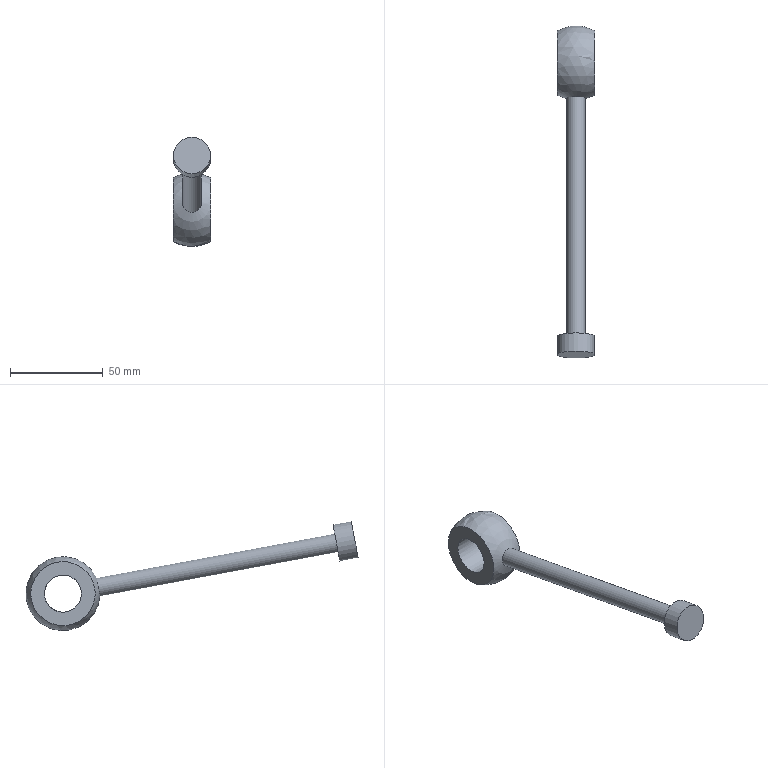Component | NX | CCJ-012 | 1 solid | 8 faces | box 20 x 179.14 x 59.02 mm | volume 30131 mm3 | plane 4 | cylinder 3 | sphere 1 | commonest cylinder face diameters 20 x2 10 x1
STEP:
#1=CARTESIAN_POINT('',(0.,0.,0.));
#2=DIRECTION('',(0.,0.,1.));
#3=DIRECTION('',(1.,0.,0.));
#4=AXIS2_PLACEMENT_3D('',#1,#2,#3);
#5=CARTESIAN_POINT('',(30.,307.867,156.612));
#6=VERTEX_POINT('',#5);
#7=CARTESIAN_POINT('',(25.,307.867,156.612));
#8=DIRECTION('',(0.,-0.9832,0.1824));
#9=DIRECTION('',(1.,0.,0.));
#10=AXIS2_PLACEMENT_3D('',#7,#8,#9);
#11=CIRCLE('',#10,5.);
#12=CARTESIAN_POINT('',(25.,326.907,153.08));
#13=DIRECTION('',(0.,0.9832,-0.1824));
#14=DIRECTION('',(1.,0.,0.));
#15=AXIS2_PLACEMENT_3D('',#12,#13,#14);
#16=SPHERICAL_SURFACE('',#15,20.);
#17=CARTESIAN_POINT('',(6.283,-1.318));
#18=CARTESIAN_POINT('',(6.188,-1.318));
#19=CARTESIAN_POINT('',(5.998,-1.318));
#20=CARTESIAN_POINT('',(5.712,-1.318));
#21=CARTESIAN_POINT('',(5.426,-1.318));
#22=CARTESIAN_POINT('',(5.141,-1.318));
#23=CARTESIAN_POINT('',(4.855,-1.318));
#24=CARTESIAN_POINT('',(4.57,-1.318));
#25=CARTESIAN_POINT('',(4.284,-1.318));
#26=CARTESIAN_POINT('',(3.998,-1.318));
#27=CARTESIAN_POINT('',(3.713,-1.318));
#28=CARTESIAN_POINT('',(3.427,-1.318));
#29=CARTESIAN_POINT('',(3.142,-1.318));
#30=CARTESIAN_POINT('',(2.856,-1.318));
#31=CARTESIAN_POINT('',(2.57,-1.318));
#32=CARTESIAN_POINT('',(2.285,-1.318));
#33=CARTESIAN_POINT('',(1.999,-1.318));
#34=CARTESIAN_POINT('',(1.714,-1.318));
#35=CARTESIAN_POINT('',(1.428,-1.318));
#36=CARTESIAN_POINT('',(1.142,-1.318));
#37=CARTESIAN_POINT('',(0.8568,-1.318));
#38=CARTESIAN_POINT('',(0.5712,-1.318));
#39=CARTESIAN_POINT('',(0.2856,-1.318));
#40=CARTESIAN_POINT('',(0.0952,-1.318));
#41=CARTESIAN_POINT('',(0.,-1.318));
#42=B_SPLINE_CURVE_WITH_KNOTS('',3,(#17,#18,#19,#20,#21,#22,#23,#24,#25,#26,#27,#28,#29,#30,#31,#32,#33,#34,#35,#36,#37,#38,#39,#40,#41),.UNSPECIFIED.,.F.,.F.,(4,1,1,1,1,1,1,1,1,1,1,1,1,1,1,1,1,1,1,1,1,1,4),(0.,0.2856,0.5712,0.8568,1.142,1.428,1.714,1.999,2.285,2.57,2.856,3.142,3.427,3.713,3.998,4.284,4.57,4.855,5.141,5.426,5.712,5.998,6.283),.QUASI_UNIFORM_KNOTS.);
#43=(GEOMETRIC_REPRESENTATION_CONTEXT(2)PARAMETRIC_REPRESENTATION_CONTEXT()REPRESENTATION_CONTEXT('',''));
#44=DEFINITIONAL_REPRESENTATION('',(#42),#43);
#45=PCURVE('',#16,#44);
#46=CARTESIAN_POINT('',(25.,179.423,180.44));
#47=DIRECTION('',(0.,0.9832,-0.1824));
#48=DIRECTION('',(1.,0.,0.));
#49=AXIS2_PLACEMENT_3D('',#46,#47,#48);
#50=CYLINDRICAL_SURFACE('',#49,5.);
#51=CARTESIAN_POINT('',(6.283,130.635));
#52=DIRECTION('',(-1.,0.));
#53=VECTOR('',#52,1.);
#54=LINE('',#51,#53);
#55=(GEOMETRIC_REPRESENTATION_CONTEXT(2)PARAMETRIC_REPRESENTATION_CONTEXT()REPRESENTATION_CONTEXT('',''));
#56=DEFINITIONAL_REPRESENTATION('',(#54),#55);
#57=PCURVE('',#50,#56);
#58=SURFACE_CURVE('',#11,(#45,#57),.PCURVE_S1.);
#59=EDGE_CURVE('',#6,#6,#58,.T.);
#60=ORIENTED_EDGE('',*,*,#59,.F.);
#61=CARTESIAN_POINT('',(35.,309.877,156.239));
#62=VERTEX_POINT('',#61);
#63=CARTESIAN_POINT('',(30.,307.867,156.612));
#64=CARTESIAN_POINT('',(31.312,308.2,156.55));
#65=CARTESIAN_POINT('',(32.593,308.649,156.467));
#66=CARTESIAN_POINT('',(33.827,309.211,156.363));
#67=CARTESIAN_POINT('',(35.,309.877,156.239));
#68=B_SPLINE_CURVE_WITH_KNOTS('',4,(#63,#64,#65,#66,#67),.UNSPECIFIED.,.F.,.F.,(5,5),(-1.318,-1.047),.PIECEWISE_BEZIER_KNOTS.);
#69=CARTESIAN_POINT('',(6.283,0.));
#70=DIRECTION('',(0.,1.));
#71=VECTOR('',#70,1.);
#72=LINE('',#69,#71);
#73=(GEOMETRIC_REPRESENTATION_CONTEXT(2)PARAMETRIC_REPRESENTATION_CONTEXT()REPRESENTATION_CONTEXT('',''));
#74=DEFINITIONAL_REPRESENTATION('',(#72),#73);
#75=PCURVE('',#16,#74);
#76=CARTESIAN_POINT('',(0.,0.));
#77=DIRECTION('',(0.,1.));
#78=VECTOR('',#77,1.);
#79=LINE('',#76,#78);
#80=(GEOMETRIC_REPRESENTATION_CONTEXT(2)PARAMETRIC_REPRESENTATION_CONTEXT()REPRESENTATION_CONTEXT('',''));
#81=DEFINITIONAL_REPRESENTATION('',(#79),#80);
#82=PCURVE('',#16,#81);
#83=SEAM_CURVE('',#68,(#75,#82),.PCURVE_S1.);
#84=EDGE_CURVE('',#6,#62,#83,.T.);
#85=ORIENTED_EDGE('',*,*,#84,.T.);
#86=CARTESIAN_POINT('',(35.,343.937,149.92));
#87=VERTEX_POINT('',#86);
#88=CARTESIAN_POINT('',(35.,326.907,153.08));
#89=DIRECTION('',(-1.,0.,0.));
#90=DIRECTION('',(0.,-0.9832,0.1824));
#91=AXIS2_PLACEMENT_3D('',#88,#89,#90);
#92=CIRCLE('',#91,17.321);
#93=CARTESIAN_POINT('',(6.283,-1.047));
#94=CARTESIAN_POINT('',(6.103,-1.047));
#95=CARTESIAN_POINT('',(5.804,-0.9974));
#96=CARTESIAN_POINT('',(5.507,-0.8234));
#97=CARTESIAN_POINT('',(5.353,-0.6063));
#98=CARTESIAN_POINT('',(5.27,-0.3694));
#99=CARTESIAN_POINT('',(5.235,-0.124));
#100=CARTESIAN_POINT('',(5.234,0.124));
#101=CARTESIAN_POINT('',(5.27,0.3694));
#102=CARTESIAN_POINT('',(5.352,0.6063));
#103=CARTESIAN_POINT('',(5.509,0.8234));
#104=CARTESIAN_POINT('',(5.796,0.9973));
#105=CARTESIAN_POINT('',(6.283,1.072));
#106=CARTESIAN_POINT('',(6.771,0.9973));
#107=CARTESIAN_POINT('',(7.057,0.8234));
#108=CARTESIAN_POINT('',(7.214,0.6063));
#109=CARTESIAN_POINT('',(7.296,0.3694));
#110=CARTESIAN_POINT('',(7.332,0.124));
#111=CARTESIAN_POINT('',(7.332,-0.124));
#112=CARTESIAN_POINT('',(7.296,-0.3694));
#113=CARTESIAN_POINT('',(7.213,-0.6063));
#114=CARTESIAN_POINT('',(7.06,-0.8234));
#115=CARTESIAN_POINT('',(6.763,-0.9974));
#116=CARTESIAN_POINT('',(6.463,-1.047));
#117=CARTESIAN_POINT('',(6.283,-1.047));
#118=B_SPLINE_CURVE_WITH_KNOTS('',3,(#93,#94,#95,#96,#97,#98,#99,#100,#101,#102,#103,#104,#105,#106,#107,#108,#109,#110,#111,#112,#113,#114,#115,#116,#117),.UNSPECIFIED.,.T.,.F.,(4,1,1,1,1,1,1,1,1,1,1,1,1,1,1,1,1,1,1,1,1,1,4),(0.,0.2856,0.5712,0.8568,1.142,1.428,1.714,1.999,2.285,2.57,2.856,3.142,3.427,3.713,3.998,4.284,4.57,4.855,5.141,5.426,5.712,5.998,6.283),.QUASI_UNIFORM_KNOTS.);
#119=(GEOMETRIC_REPRESENTATION_CONTEXT(2)PARAMETRIC_REPRESENTATION_CONTEXT()REPRESENTATION_CONTEXT('',''));
#120=DEFINITIONAL_REPRESENTATION('',(#118),#119);
#121=PCURVE('',#16,#120);
#122=CARTESIAN_POINT('',(35.,179.423,180.44));
#123=DIRECTION('',(1.,0.,0.));
#124=DIRECTION('',(0.,-0.9832,0.1824));
#125=AXIS2_PLACEMENT_3D('',#122,#123,#124);
#126=PLANE('',#125);
#127=CARTESIAN_POINT('',(-132.679,-0.));
#128=CARTESIAN_POINT('',(-132.679,-30.));
#129=CARTESIAN_POINT('',(-158.66,-15.));
#130=CARTESIAN_POINT('',(-184.641,-0.));
#131=CARTESIAN_POINT('',(-158.66,15.));
#132=CARTESIAN_POINT('',(-132.679,30.));
#133=CARTESIAN_POINT('',(-132.679,-0.));
#134=(BOUNDED_CURVE()B_SPLINE_CURVE(2,(#127,#128,#129,#130,#131,#132,#133),.UNSPECIFIED.,.T.,.F.)B_SPLINE_CURVE_WITH_KNOTS((1,2,2,2,2,1),(-2.094,0.,2.094,4.189,6.283,8.378),.UNSPECIFIED.)CURVE()GEOMETRIC_REPRESENTATION_ITEM()RATIONAL_B_SPLINE_CURVE((1.,0.5,1.,0.5,1.,0.5,1.))REPRESENTATION_ITEM(''));
#135=(GEOMETRIC_REPRESENTATION_CONTEXT(2)PARAMETRIC_REPRESENTATION_CONTEXT()REPRESENTATION_CONTEXT('',''));
#136=DEFINITIONAL_REPRESENTATION('',(#134),#135);
#137=PCURVE('',#126,#136);
#138=SURFACE_CURVE('',#92,(#121,#137),.PCURVE_S1.);
#139=EDGE_CURVE('',#62,#87,#138,.T.);
#140=ORIENTED_EDGE('',*,*,#139,.T.);
#141=CARTESIAN_POINT('',(25.,346.571,149.432));
#142=VERTEX_POINT('',#141);
#143=CARTESIAN_POINT('',(35.,343.937,149.92));
#144=CARTESIAN_POINT('',(33.186,344.966,149.729));
#145=CARTESIAN_POINT('',(31.235,345.763,149.582));
#146=CARTESIAN_POINT('',(29.189,346.302,149.482));
#147=CARTESIAN_POINT('',(27.094,346.571,149.432));
#148=CARTESIAN_POINT('',(25.,346.571,149.432));
#149=B_SPLINE_CURVE_WITH_KNOTS('',5,(#143,#144,#145,#146,#147,#148),.UNSPECIFIED.,.F.,.F.,(6,6),(1.047,1.571),.PIECEWISE_BEZIER_KNOTS.);
#150=CARTESIAN_POINT('',(6.283,0.));
#151=DIRECTION('',(0.,1.));
#152=VECTOR('',#151,1.);
#153=LINE('',#150,#152);
#154=(GEOMETRIC_REPRESENTATION_CONTEXT(2)PARAMETRIC_REPRESENTATION_CONTEXT()REPRESENTATION_CONTEXT('',''));
#155=DEFINITIONAL_REPRESENTATION('',(#153),#154);
#156=PCURVE('',#16,#155);
#157=CARTESIAN_POINT('',(0.,0.));
#158=DIRECTION('',(0.,1.));
#159=VECTOR('',#158,1.);
#160=LINE('',#157,#159);
#161=(GEOMETRIC_REPRESENTATION_CONTEXT(2)PARAMETRIC_REPRESENTATION_CONTEXT()REPRESENTATION_CONTEXT('',''));
#162=DEFINITIONAL_REPRESENTATION('',(#160),#161);
#163=PCURVE('',#16,#162);
#164=SEAM_CURVE('',#149,(#156,#163),.PCURVE_S1.);
#165=EDGE_CURVE('',#87,#142,#164,.T.);
#166=ORIENTED_EDGE('',*,*,#165,.T.);
#167=ORIENTED_EDGE('',*,*,#165,.F.);
#168=CARTESIAN_POINT('',(35.,326.907,153.08));
#169=DIRECTION('',(-1.,0.,0.));
#170=DIRECTION('',(0.,-0.9832,0.1824));
#171=AXIS2_PLACEMENT_3D('',#168,#169,#170);
#172=CIRCLE('',#171,17.321);
#173=CARTESIAN_POINT('',(-0.,-1.047));
#174=CARTESIAN_POINT('',(-0.1797,-1.047));
#175=CARTESIAN_POINT('',(-0.4794,-0.9974));
#176=CARTESIAN_POINT('',(-0.7765,-0.8234));
#177=CARTESIAN_POINT('',(-0.9302,-0.6063));
#178=CARTESIAN_POINT('',(-1.013,-0.3694));
#179=CARTESIAN_POINT('',(-1.049,-0.124));
#180=CARTESIAN_POINT('',(-1.049,0.124));
#181=CARTESIAN_POINT('',(-1.013,0.3694));
#182=CARTESIAN_POINT('',(-0.9308,0.6063));
#183=CARTESIAN_POINT('',(-0.7743,0.8234));
#184=CARTESIAN_POINT('',(-0.4874,0.9973));
#185=CARTESIAN_POINT('',(0.,1.072));
#186=CARTESIAN_POINT('',(0.4874,0.9973));
#187=CARTESIAN_POINT('',(0.7743,0.8234));
#188=CARTESIAN_POINT('',(0.9308,0.6063));
#189=CARTESIAN_POINT('',(1.013,0.3694));
#190=CARTESIAN_POINT('',(1.049,0.124));
#191=CARTESIAN_POINT('',(1.049,-0.124));
#192=CARTESIAN_POINT('',(1.013,-0.3694));
#193=CARTESIAN_POINT('',(0.9302,-0.6063));
#194=CARTESIAN_POINT('',(0.7765,-0.8234));
#195=CARTESIAN_POINT('',(0.4794,-0.9974));
#196=CARTESIAN_POINT('',(0.1797,-1.047));
#197=CARTESIAN_POINT('',(-0.,-1.047));
#198=B_SPLINE_CURVE_WITH_KNOTS('',3,(#173,#174,#175,#176,#177,#178,#179,#180,#181,#182,#183,#184,#185,#186,#187,#188,#189,#190,#191,#192,#193,#194,#195,#196,#197),.UNSPECIFIED.,.T.,.F.,(4,1,1,1,1,1,1,1,1,1,1,1,1,1,1,1,1,1,1,1,1,1,4),(0.,0.2856,0.5712,0.8568,1.142,1.428,1.714,1.999,2.285,2.57,2.856,3.142,3.427,3.713,3.998,4.284,4.57,4.855,5.141,5.426,5.712,5.998,6.283),.QUASI_UNIFORM_KNOTS.);
#199=(GEOMETRIC_REPRESENTATION_CONTEXT(2)PARAMETRIC_REPRESENTATION_CONTEXT()REPRESENTATION_CONTEXT('',''));
#200=DEFINITIONAL_REPRESENTATION('',(#198),#199);
#201=PCURVE('',#16,#200);
#202=CARTESIAN_POINT('',(-132.679,-0.));
#203=CARTESIAN_POINT('',(-132.679,-30.));
#204=CARTESIAN_POINT('',(-158.66,-15.));
#205=CARTESIAN_POINT('',(-184.641,-0.));
#206=CARTESIAN_POINT('',(-158.66,15.));
#207=CARTESIAN_POINT('',(-132.679,30.));
#208=CARTESIAN_POINT('',(-132.679,-0.));
#209=(BOUNDED_CURVE()B_SPLINE_CURVE(2,(#202,#203,#204,#205,#206,#207,#208),.UNSPECIFIED.,.T.,.F.)B_SPLINE_CURVE_WITH_KNOTS((1,2,2,2,2,1),(-2.094,0.,2.094,4.189,6.283,8.378),.UNSPECIFIED.)CURVE()GEOMETRIC_REPRESENTATION_ITEM()RATIONAL_B_SPLINE_CURVE((1.,0.5,1.,0.5,1.,0.5,1.))REPRESENTATION_ITEM(''));
#210=(GEOMETRIC_REPRESENTATION_CONTEXT(2)PARAMETRIC_REPRESENTATION_CONTEXT()REPRESENTATION_CONTEXT('',''));
#211=DEFINITIONAL_REPRESENTATION('',(#209),#210);
#212=PCURVE('',#126,#211);
#213=SURFACE_CURVE('',#172,(#201,#212),.PCURVE_S1.);
#214=EDGE_CURVE('',#87,#62,#213,.T.);
#215=ORIENTED_EDGE('',*,*,#214,.T.);
#216=ORIENTED_EDGE('',*,*,#84,.F.);
#217=EDGE_LOOP('',(#60,#85,#140,#166,#167,#215,#216));
#218=FACE_BOUND('',#217,.T.);
#219=CARTESIAN_POINT('',(15.,343.937,149.92));
#220=VERTEX_POINT('',#219);
#221=CARTESIAN_POINT('',(15.,326.907,153.08));
#222=DIRECTION('',(1.,0.,0.));
#223=DIRECTION('',(0.,0.9832,-0.1824));
#224=AXIS2_PLACEMENT_3D('',#221,#222,#223);
#225=CIRCLE('',#224,17.321);
#226=CARTESIAN_POINT('',(3.142,1.047));
#227=CARTESIAN_POINT('',(3.321,1.047));
#228=CARTESIAN_POINT('',(3.621,0.9974));
#229=CARTESIAN_POINT('',(3.918,0.8234));
#230=CARTESIAN_POINT('',(4.072,0.6063));
#231=CARTESIAN_POINT('',(4.155,0.3694));
#232=CARTESIAN_POINT('',(4.19,0.124));
#233=CARTESIAN_POINT('',(4.19,-0.124));
#234=CARTESIAN_POINT('',(4.155,-0.3694));
#235=CARTESIAN_POINT('',(4.072,-0.6063));
#236=CARTESIAN_POINT('',(3.916,-0.8234));
#237=CARTESIAN_POINT('',(3.629,-0.9973));
#238=CARTESIAN_POINT('',(3.142,-1.072));
#239=CARTESIAN_POINT('',(2.654,-0.9973));
#240=CARTESIAN_POINT('',(2.367,-0.8234));
#241=CARTESIAN_POINT('',(2.211,-0.6063));
#242=CARTESIAN_POINT('',(2.129,-0.3694));
#243=CARTESIAN_POINT('',(2.093,-0.124));
#244=CARTESIAN_POINT('',(2.093,0.124));
#245=CARTESIAN_POINT('',(2.128,0.3694));
#246=CARTESIAN_POINT('',(2.211,0.6063));
#247=CARTESIAN_POINT('',(2.365,0.8234));
#248=CARTESIAN_POINT('',(2.662,0.9974));
#249=CARTESIAN_POINT('',(2.962,1.047));
#250=CARTESIAN_POINT('',(3.142,1.047));
#251=B_SPLINE_CURVE_WITH_KNOTS('',3,(#226,#227,#228,#229,#230,#231,#232,#233,#234,#235,#236,#237,#238,#239,#240,#241,#242,#243,#244,#245,#246,#247,#248,#249,#250),.UNSPECIFIED.,.T.,.F.,(4,1,1,1,1,1,1,1,1,1,1,1,1,1,1,1,1,1,1,1,1,1,4),(0.,0.2856,0.5712,0.8568,1.142,1.428,1.714,1.999,2.285,2.57,2.856,3.142,3.427,3.713,3.998,4.284,4.57,4.855,5.141,5.426,5.712,5.998,6.283),.QUASI_UNIFORM_KNOTS.);
#252=(GEOMETRIC_REPRESENTATION_CONTEXT(2)PARAMETRIC_REPRESENTATION_CONTEXT()REPRESENTATION_CONTEXT('',''));
#253=DEFINITIONAL_REPRESENTATION('',(#251),#252);
#254=PCURVE('',#16,#253);
#255=CARTESIAN_POINT('',(15.,179.423,180.44));
#256=DIRECTION('',(-1.,0.,0.));
#257=DIRECTION('',(0.,0.9832,-0.1824));
#258=AXIS2_PLACEMENT_3D('',#255,#256,#257);
#259=PLANE('',#258);
#260=CARTESIAN_POINT('',(167.321,-0.));
#261=CARTESIAN_POINT('',(167.321,-30.));
#262=CARTESIAN_POINT('',(141.34,-15.));
#263=CARTESIAN_POINT('',(115.359,-0.));
#264=CARTESIAN_POINT('',(141.34,15.));
#265=CARTESIAN_POINT('',(167.321,30.));
#266=CARTESIAN_POINT('',(167.321,-0.));
#267=(BOUNDED_CURVE()B_SPLINE_CURVE(2,(#260,#261,#262,#263,#264,#265,#266),.UNSPECIFIED.,.T.,.F.)B_SPLINE_CURVE_WITH_KNOTS((1,2,2,2,2,1),(-2.094,0.,2.094,4.189,6.283,8.378),.UNSPECIFIED.)CURVE()GEOMETRIC_REPRESENTATION_ITEM()RATIONAL_B_SPLINE_CURVE((1.,0.5,1.,0.5,1.,0.5,1.))REPRESENTATION_ITEM(''));
#268=(GEOMETRIC_REPRESENTATION_CONTEXT(2)PARAMETRIC_REPRESENTATION_CONTEXT()REPRESENTATION_CONTEXT('',''));
#269=DEFINITIONAL_REPRESENTATION('',(#267),#268);
#270=PCURVE('',#259,#269);
#271=SURFACE_CURVE('',#225,(#254,#270),.PCURVE_S1.);
#272=EDGE_CURVE('',#220,#220,#271,.T.);
#273=ORIENTED_EDGE('',*,*,#272,.T.);
#274=EDGE_LOOP('',(#273));
#275=FACE_BOUND('',#274,.T.);
#276=ADVANCED_FACE('',(#218,#275),#16,.T.);
#277=ORIENTED_EDGE('',*,*,#59,.T.);
#278=CARTESIAN_POINT('',(30.,179.423,180.44));
#279=VERTEX_POINT('',#278);
#280=CARTESIAN_POINT('',(30.,179.423,180.44));
#281=CARTESIAN_POINT('',(30.,307.867,156.612));
#282=B_SPLINE_CURVE_WITH_KNOTS('',1,(#280,#281),.UNSPECIFIED.,.F.,.F.,(2,2),(0.,130.635),.PIECEWISE_BEZIER_KNOTS.);
#283=CARTESIAN_POINT('',(0.,0.));
#284=DIRECTION('',(0.,1.));
#285=VECTOR('',#284,1.);
#286=LINE('',#283,#285);
#287=(GEOMETRIC_REPRESENTATION_CONTEXT(2)PARAMETRIC_REPRESENTATION_CONTEXT()REPRESENTATION_CONTEXT('',''));
#288=DEFINITIONAL_REPRESENTATION('',(#286),#287);
#289=PCURVE('',#50,#288);
#290=CARTESIAN_POINT('',(6.283,0.));
#291=DIRECTION('',(0.,1.));
#292=VECTOR('',#291,1.);
#293=LINE('',#290,#292);
#294=(GEOMETRIC_REPRESENTATION_CONTEXT(2)PARAMETRIC_REPRESENTATION_CONTEXT()REPRESENTATION_CONTEXT('',''));
#295=DEFINITIONAL_REPRESENTATION('',(#293),#294);
#296=PCURVE('',#50,#295);
#297=SEAM_CURVE('',#282,(#289,#296),.PCURVE_S1.);
#298=EDGE_CURVE('',#279,#6,#297,.T.);
#299=ORIENTED_EDGE('',*,*,#298,.F.);
#300=CARTESIAN_POINT('',(25.,179.423,180.44));
#301=DIRECTION('',(0.,0.9832,-0.1824));
#302=DIRECTION('',(1.,0.,0.));
#303=AXIS2_PLACEMENT_3D('',#300,#301,#302);
#304=CIRCLE('',#303,5.);
#305=CARTESIAN_POINT('',(0.,0.));
#306=DIRECTION('',(1.,0.));
#307=VECTOR('',#306,1.);
#308=LINE('',#305,#307);
#309=(GEOMETRIC_REPRESENTATION_CONTEXT(2)PARAMETRIC_REPRESENTATION_CONTEXT()REPRESENTATION_CONTEXT('',''));
#310=DEFINITIONAL_REPRESENTATION('',(#308),#309);
#311=PCURVE('',#50,#310);
#312=CARTESIAN_POINT('',(25.,179.423,180.44));
#313=DIRECTION('',(0.,-0.9832,0.1824));
#314=DIRECTION('',(-1.,0.,0.));
#315=AXIS2_PLACEMENT_3D('',#312,#313,#314);
#316=PLANE('',#315);
#317=CARTESIAN_POINT('',(-5.,0.));
#318=CARTESIAN_POINT('',(-5.,8.66));
#319=CARTESIAN_POINT('',(2.5,4.33));
#320=CARTESIAN_POINT('',(10.,0.));
#321=CARTESIAN_POINT('',(2.5,-4.33));
#322=CARTESIAN_POINT('',(-5.,-8.66));
#323=CARTESIAN_POINT('',(-5.,0.));
#324=(BOUNDED_CURVE()B_SPLINE_CURVE(2,(#317,#318,#319,#320,#321,#322,#323),.UNSPECIFIED.,.T.,.F.)B_SPLINE_CURVE_WITH_KNOTS((1,2,2,2,2,1),(-2.094,0.,2.094,4.189,6.283,8.378),.UNSPECIFIED.)CURVE()GEOMETRIC_REPRESENTATION_ITEM()RATIONAL_B_SPLINE_CURVE((1.,0.5,1.,0.5,1.,0.5,1.))REPRESENTATION_ITEM(''));
#325=(GEOMETRIC_REPRESENTATION_CONTEXT(2)PARAMETRIC_REPRESENTATION_CONTEXT()REPRESENTATION_CONTEXT('',''));
#326=DEFINITIONAL_REPRESENTATION('',(#324),#325);
#327=PCURVE('',#316,#326);
#328=SURFACE_CURVE('',#304,(#311,#327),.PCURVE_S1.);
#329=EDGE_CURVE('',#279,#279,#328,.T.);
#330=ORIENTED_EDGE('',*,*,#329,.T.);
#331=ORIENTED_EDGE('',*,*,#298,.T.);
#332=EDGE_LOOP('',(#277,#299,#330,#331));
#333=FACE_BOUND('',#332,.T.);
#334=ADVANCED_FACE('',(#333),#50,.T.);
#335=CARTESIAN_POINT('',(15.,336.739,151.256));
#336=VERTEX_POINT('',#335);
#337=CARTESIAN_POINT('',(15.,325.083,143.247));
#338=VERTEX_POINT('',#337);
#339=CARTESIAN_POINT('',(15.,326.907,153.08));
#340=DIRECTION('',(-1.,0.,0.));
#341=DIRECTION('',(0.,0.9832,-0.1824));
#342=AXIS2_PLACEMENT_3D('',#339,#340,#341);
#343=CIRCLE('',#342,10.);
#344=CARTESIAN_POINT('',(150.,0.));
#345=DIRECTION('',(1.,0.));
#346=AXIS2_PLACEMENT_2D('',#344,#345);
#347=CIRCLE('',#346,10.);
#348=(GEOMETRIC_REPRESENTATION_CONTEXT(2)PARAMETRIC_REPRESENTATION_CONTEXT()REPRESENTATION_CONTEXT('',''));
#349=DEFINITIONAL_REPRESENTATION('',(#347),#348);
#350=PCURVE('',#259,#349);
#351=CARTESIAN_POINT('',(-25.,326.907,153.08));
#352=DIRECTION('',(1.,0.,0.));
#353=DIRECTION('',(0.,-0.9832,0.1824));
#354=AXIS2_PLACEMENT_3D('',#351,#352,#353);
#355=CYLINDRICAL_SURFACE('',#354,10.);
#356=CARTESIAN_POINT('',(3.142,40.));
#357=DIRECTION('',(-1.,0.));
#358=VECTOR('',#357,1.);
#359=LINE('',#356,#358);
#360=(GEOMETRIC_REPRESENTATION_CONTEXT(2)PARAMETRIC_REPRESENTATION_CONTEXT()REPRESENTATION_CONTEXT('',''));
#361=DEFINITIONAL_REPRESENTATION('',(#359),#360);
#362=PCURVE('',#355,#361);
#363=SURFACE_CURVE('',#343,(#350,#362),.PCURVE_S1.);
#364=EDGE_CURVE('',#336,#338,#363,.T.);
#365=ORIENTED_EDGE('',*,*,#364,.F.);
#366=CARTESIAN_POINT('',(15.,326.907,153.08));
#367=DIRECTION('',(-1.,0.,0.));
#368=DIRECTION('',(0.,0.9832,-0.1824));
#369=AXIS2_PLACEMENT_3D('',#366,#367,#368);
#370=CIRCLE('',#369,10.);
#371=CARTESIAN_POINT('',(150.,0.));
#372=DIRECTION('',(1.,0.));
#373=AXIS2_PLACEMENT_2D('',#371,#372);
#374=CIRCLE('',#373,10.);
#375=(GEOMETRIC_REPRESENTATION_CONTEXT(2)PARAMETRIC_REPRESENTATION_CONTEXT()REPRESENTATION_CONTEXT('',''));
#376=DEFINITIONAL_REPRESENTATION('',(#374),#375);
#377=PCURVE('',#259,#376);
#378=CARTESIAN_POINT('',(9.425,40.));
#379=DIRECTION('',(-1.,0.));
#380=VECTOR('',#379,1.);
#381=LINE('',#378,#380);
#382=(GEOMETRIC_REPRESENTATION_CONTEXT(2)PARAMETRIC_REPRESENTATION_CONTEXT()REPRESENTATION_CONTEXT('',''));
#383=DEFINITIONAL_REPRESENTATION('',(#381),#382);
#384=PCURVE('',#355,#383);
#385=SURFACE_CURVE('',#370,(#377,#384),.PCURVE_S1.);
#386=EDGE_CURVE('',#338,#336,#385,.T.);
#387=ORIENTED_EDGE('',*,*,#386,.F.);
#388=EDGE_LOOP('',(#365,#387));
#389=FACE_BOUND('',#388,.T.);
#390=ORIENTED_EDGE('',*,*,#272,.F.);
#391=EDGE_LOOP('',(#390));
#392=FACE_BOUND('',#391,.T.);
#393=ADVANCED_FACE('',(#389,#392),#259,.T.);
#394=CARTESIAN_POINT('',(35.,325.083,143.247));
#395=VERTEX_POINT('',#394);
#396=CARTESIAN_POINT('',(35.,326.907,153.08));
#397=DIRECTION('',(1.,0.,0.));
#398=DIRECTION('',(0.,-0.1824,-0.9832));
#399=AXIS2_PLACEMENT_3D('',#396,#397,#398);
#400=CIRCLE('',#399,10.);
#401=CARTESIAN_POINT('',(-150.,0.));
#402=DIRECTION('',(-0.,1.));
#403=AXIS2_PLACEMENT_2D('',#401,#402);
#404=CIRCLE('',#403,10.);
#405=(GEOMETRIC_REPRESENTATION_CONTEXT(2)PARAMETRIC_REPRESENTATION_CONTEXT()REPRESENTATION_CONTEXT('',''));
#406=DEFINITIONAL_REPRESENTATION('',(#404),#405);
#407=PCURVE('',#126,#406);
#408=CARTESIAN_POINT('',(1.571,60.));
#409=DIRECTION('',(1.,0.));
#410=VECTOR('',#409,1.);
#411=LINE('',#408,#410);
#412=(GEOMETRIC_REPRESENTATION_CONTEXT(2)PARAMETRIC_REPRESENTATION_CONTEXT()REPRESENTATION_CONTEXT('',''));
#413=DEFINITIONAL_REPRESENTATION('',(#411),#412);
#414=PCURVE('',#355,#413);
#415=SURFACE_CURVE('',#400,(#407,#414),.PCURVE_S1.);
#416=EDGE_CURVE('',#395,#395,#415,.T.);
#417=ORIENTED_EDGE('',*,*,#416,.F.);
#418=EDGE_LOOP('',(#417));
#419=FACE_BOUND('',#418,.T.);
#420=ORIENTED_EDGE('',*,*,#139,.F.);
#421=ORIENTED_EDGE('',*,*,#214,.F.);
#422=EDGE_LOOP('',(#420,#421));
#423=FACE_BOUND('',#422,.T.);
#424=ADVANCED_FACE('',(#419,#423),#126,.T.);
#425=ORIENTED_EDGE('',*,*,#386,.F.);
#426=CARTESIAN_POINT('',(15.,325.083,143.247));
#427=CARTESIAN_POINT('',(35.,325.083,143.247));
#428=B_SPLINE_CURVE_WITH_KNOTS('',1,(#426,#427),.UNSPECIFIED.,.F.,.F.,(2,2),(40.,60.),.PIECEWISE_BEZIER_KNOTS.);
#429=CARTESIAN_POINT('',(7.854,0.));
#430=DIRECTION('',(0.,1.));
#431=VECTOR('',#430,1.);
#432=LINE('',#429,#431);
#433=(GEOMETRIC_REPRESENTATION_CONTEXT(2)PARAMETRIC_REPRESENTATION_CONTEXT()REPRESENTATION_CONTEXT('',''));
#434=DEFINITIONAL_REPRESENTATION('',(#432),#433);
#435=PCURVE('',#355,#434);
#436=CARTESIAN_POINT('',(1.571,0.));
#437=DIRECTION('',(0.,1.));
#438=VECTOR('',#437,1.);
#439=LINE('',#436,#438);
#440=(GEOMETRIC_REPRESENTATION_CONTEXT(2)PARAMETRIC_REPRESENTATION_CONTEXT()REPRESENTATION_CONTEXT('',''));
#441=DEFINITIONAL_REPRESENTATION('',(#439),#440);
#442=PCURVE('',#355,#441);
#443=SEAM_CURVE('',#428,(#435,#442),.PCURVE_S1.);
#444=EDGE_CURVE('',#338,#395,#443,.T.);
#445=ORIENTED_EDGE('',*,*,#444,.T.);
#446=ORIENTED_EDGE('',*,*,#416,.F.);
#447=ORIENTED_EDGE('',*,*,#444,.F.);
#448=ORIENTED_EDGE('',*,*,#364,.F.);
#449=EDGE_LOOP('',(#425,#445,#446,#447,#448));
#450=FACE_BOUND('',#449,.F.);
#451=ADVANCED_FACE('',(#450),#355,.F.);
#452=CARTESIAN_POINT('',(15.,169.591,182.264));
#453=VERTEX_POINT('',#452);
#454=CARTESIAN_POINT('',(25.,169.591,182.264));
#455=DIRECTION('',(0.,-0.9832,0.1824));
#456=DIRECTION('',(-1.,0.,0.));
#457=AXIS2_PLACEMENT_3D('',#454,#455,#456);
#458=CIRCLE('',#457,10.);
#459=CARTESIAN_POINT('',(25.,169.591,182.264));
#460=DIRECTION('',(0.,0.9832,-0.1824));
#461=DIRECTION('',(1.,0.,0.));
#462=AXIS2_PLACEMENT_3D('',#459,#460,#461);
#463=CYLINDRICAL_SURFACE('',#462,10.);
#464=CARTESIAN_POINT('',(9.425,0.));
#465=DIRECTION('',(-1.,0.));
#466=VECTOR('',#465,1.);
#467=LINE('',#464,#466);
#468=(GEOMETRIC_REPRESENTATION_CONTEXT(2)PARAMETRIC_REPRESENTATION_CONTEXT()REPRESENTATION_CONTEXT('',''));
#469=DEFINITIONAL_REPRESENTATION('',(#467),#468);
#470=PCURVE('',#463,#469);
#471=CARTESIAN_POINT('',(25.,169.591,182.264));
#472=DIRECTION('',(0.,-0.9832,0.1824));
#473=DIRECTION('',(-1.,0.,0.));
#474=AXIS2_PLACEMENT_3D('',#471,#472,#473);
#475=PLANE('',#474);
#476=CARTESIAN_POINT('',(0.,0.));
#477=DIRECTION('',(1.,0.));
#478=AXIS2_PLACEMENT_2D('',#476,#477);
#479=CIRCLE('',#478,10.);
#480=(GEOMETRIC_REPRESENTATION_CONTEXT(2)PARAMETRIC_REPRESENTATION_CONTEXT()REPRESENTATION_CONTEXT('',''));
#481=DEFINITIONAL_REPRESENTATION('',(#479),#480);
#482=PCURVE('',#475,#481);
#483=SURFACE_CURVE('',#458,(#470,#482),.PCURVE_S1.);
#484=EDGE_CURVE('',#453,#453,#483,.T.);
#485=ORIENTED_EDGE('',*,*,#484,.F.);
#486=CARTESIAN_POINT('',(15.,179.423,180.44));
#487=VERTEX_POINT('',#486);
#488=CARTESIAN_POINT('',(15.,169.591,182.264));
#489=CARTESIAN_POINT('',(15.,179.423,180.44));
#490=B_SPLINE_CURVE_WITH_KNOTS('',1,(#488,#489),.UNSPECIFIED.,.F.,.F.,(2,2),(0.,10.),.PIECEWISE_BEZIER_KNOTS.);
#491=CARTESIAN_POINT('',(9.425,0.));
#492=DIRECTION('',(0.,1.));
#493=VECTOR('',#492,1.);
#494=LINE('',#491,#493);
#495=(GEOMETRIC_REPRESENTATION_CONTEXT(2)PARAMETRIC_REPRESENTATION_CONTEXT()REPRESENTATION_CONTEXT('',''));
#496=DEFINITIONAL_REPRESENTATION('',(#494),#495);
#497=PCURVE('',#463,#496);
#498=CARTESIAN_POINT('',(3.142,0.));
#499=DIRECTION('',(0.,1.));
#500=VECTOR('',#499,1.);
#501=LINE('',#498,#500);
#502=(GEOMETRIC_REPRESENTATION_CONTEXT(2)PARAMETRIC_REPRESENTATION_CONTEXT()REPRESENTATION_CONTEXT('',''));
#503=DEFINITIONAL_REPRESENTATION('',(#501),#502);
#504=PCURVE('',#463,#503);
#505=SEAM_CURVE('',#490,(#497,#504),.PCURVE_S1.);
#506=EDGE_CURVE('',#453,#487,#505,.T.);
#507=ORIENTED_EDGE('',*,*,#506,.T.);
#508=CARTESIAN_POINT('',(25.,179.423,180.44));
#509=DIRECTION('',(0.,-0.9832,0.1824));
#510=DIRECTION('',(-1.,0.,0.));
#511=AXIS2_PLACEMENT_3D('',#508,#509,#510);
#512=CIRCLE('',#511,10.);
#513=CARTESIAN_POINT('',(9.425,10.));
#514=DIRECTION('',(-1.,0.));
#515=VECTOR('',#514,1.);
#516=LINE('',#513,#515);
#517=(GEOMETRIC_REPRESENTATION_CONTEXT(2)PARAMETRIC_REPRESENTATION_CONTEXT()REPRESENTATION_CONTEXT('',''));
#518=DEFINITIONAL_REPRESENTATION('',(#516),#517);
#519=PCURVE('',#463,#518);
#520=CARTESIAN_POINT('',(0.,0.));
#521=DIRECTION('',(1.,0.));
#522=AXIS2_PLACEMENT_2D('',#520,#521);
#523=CIRCLE('',#522,10.);
#524=(GEOMETRIC_REPRESENTATION_CONTEXT(2)PARAMETRIC_REPRESENTATION_CONTEXT()REPRESENTATION_CONTEXT('',''));
#525=DEFINITIONAL_REPRESENTATION('',(#523),#524);
#526=PCURVE('',#316,#525);
#527=SURFACE_CURVE('',#512,(#519,#526),.PCURVE_S1.);
#528=EDGE_CURVE('',#487,#487,#527,.T.);
#529=ORIENTED_EDGE('',*,*,#528,.T.);
#530=ORIENTED_EDGE('',*,*,#506,.F.);
#531=EDGE_LOOP('',(#485,#507,#529,#530));
#532=FACE_BOUND('',#531,.T.);
#533=ADVANCED_FACE('',(#532),#463,.T.);
#534=ORIENTED_EDGE('',*,*,#484,.T.);
#535=EDGE_LOOP('',(#534));
#536=FACE_BOUND('',#535,.T.);
#537=ADVANCED_FACE('',(#536),#475,.T.);
#538=ORIENTED_EDGE('',*,*,#329,.F.);
#539=EDGE_LOOP('',(#538));
#540=FACE_BOUND('',#539,.T.);
#541=ORIENTED_EDGE('',*,*,#528,.F.);
#542=EDGE_LOOP('',(#541));
#543=FACE_BOUND('',#542,.T.);
#544=ADVANCED_FACE('',(#540,#543),#316,.F.);
#545=CLOSED_SHELL('',(#276,#334,#393,#424,#451,#533,#537,#544));
#546=MANIFOLD_SOLID_BREP('',#545);
#547=(LENGTH_UNIT()NAMED_UNIT(*)SI_UNIT(.MILLI.,.METRE.));
#548=UNCERTAINTY_MEASURE_WITH_UNIT(LENGTH_MEASURE(0.01),#547,'','');
#549=(NAMED_UNIT(*)PLANE_ANGLE_UNIT()SI_UNIT($,.RADIAN.));
#550=(NAMED_UNIT(*)SI_UNIT($,.STERADIAN.)SOLID_ANGLE_UNIT());
#551=(GEOMETRIC_REPRESENTATION_CONTEXT(3)GLOBAL_UNCERTAINTY_ASSIGNED_CONTEXT((#548))GLOBAL_UNIT_ASSIGNED_CONTEXT((#547,#549,#550))REPRESENTATION_CONTEXT('',''));
#552=ADVANCED_BREP_SHAPE_REPRESENTATION('',(#4,#546),#551);